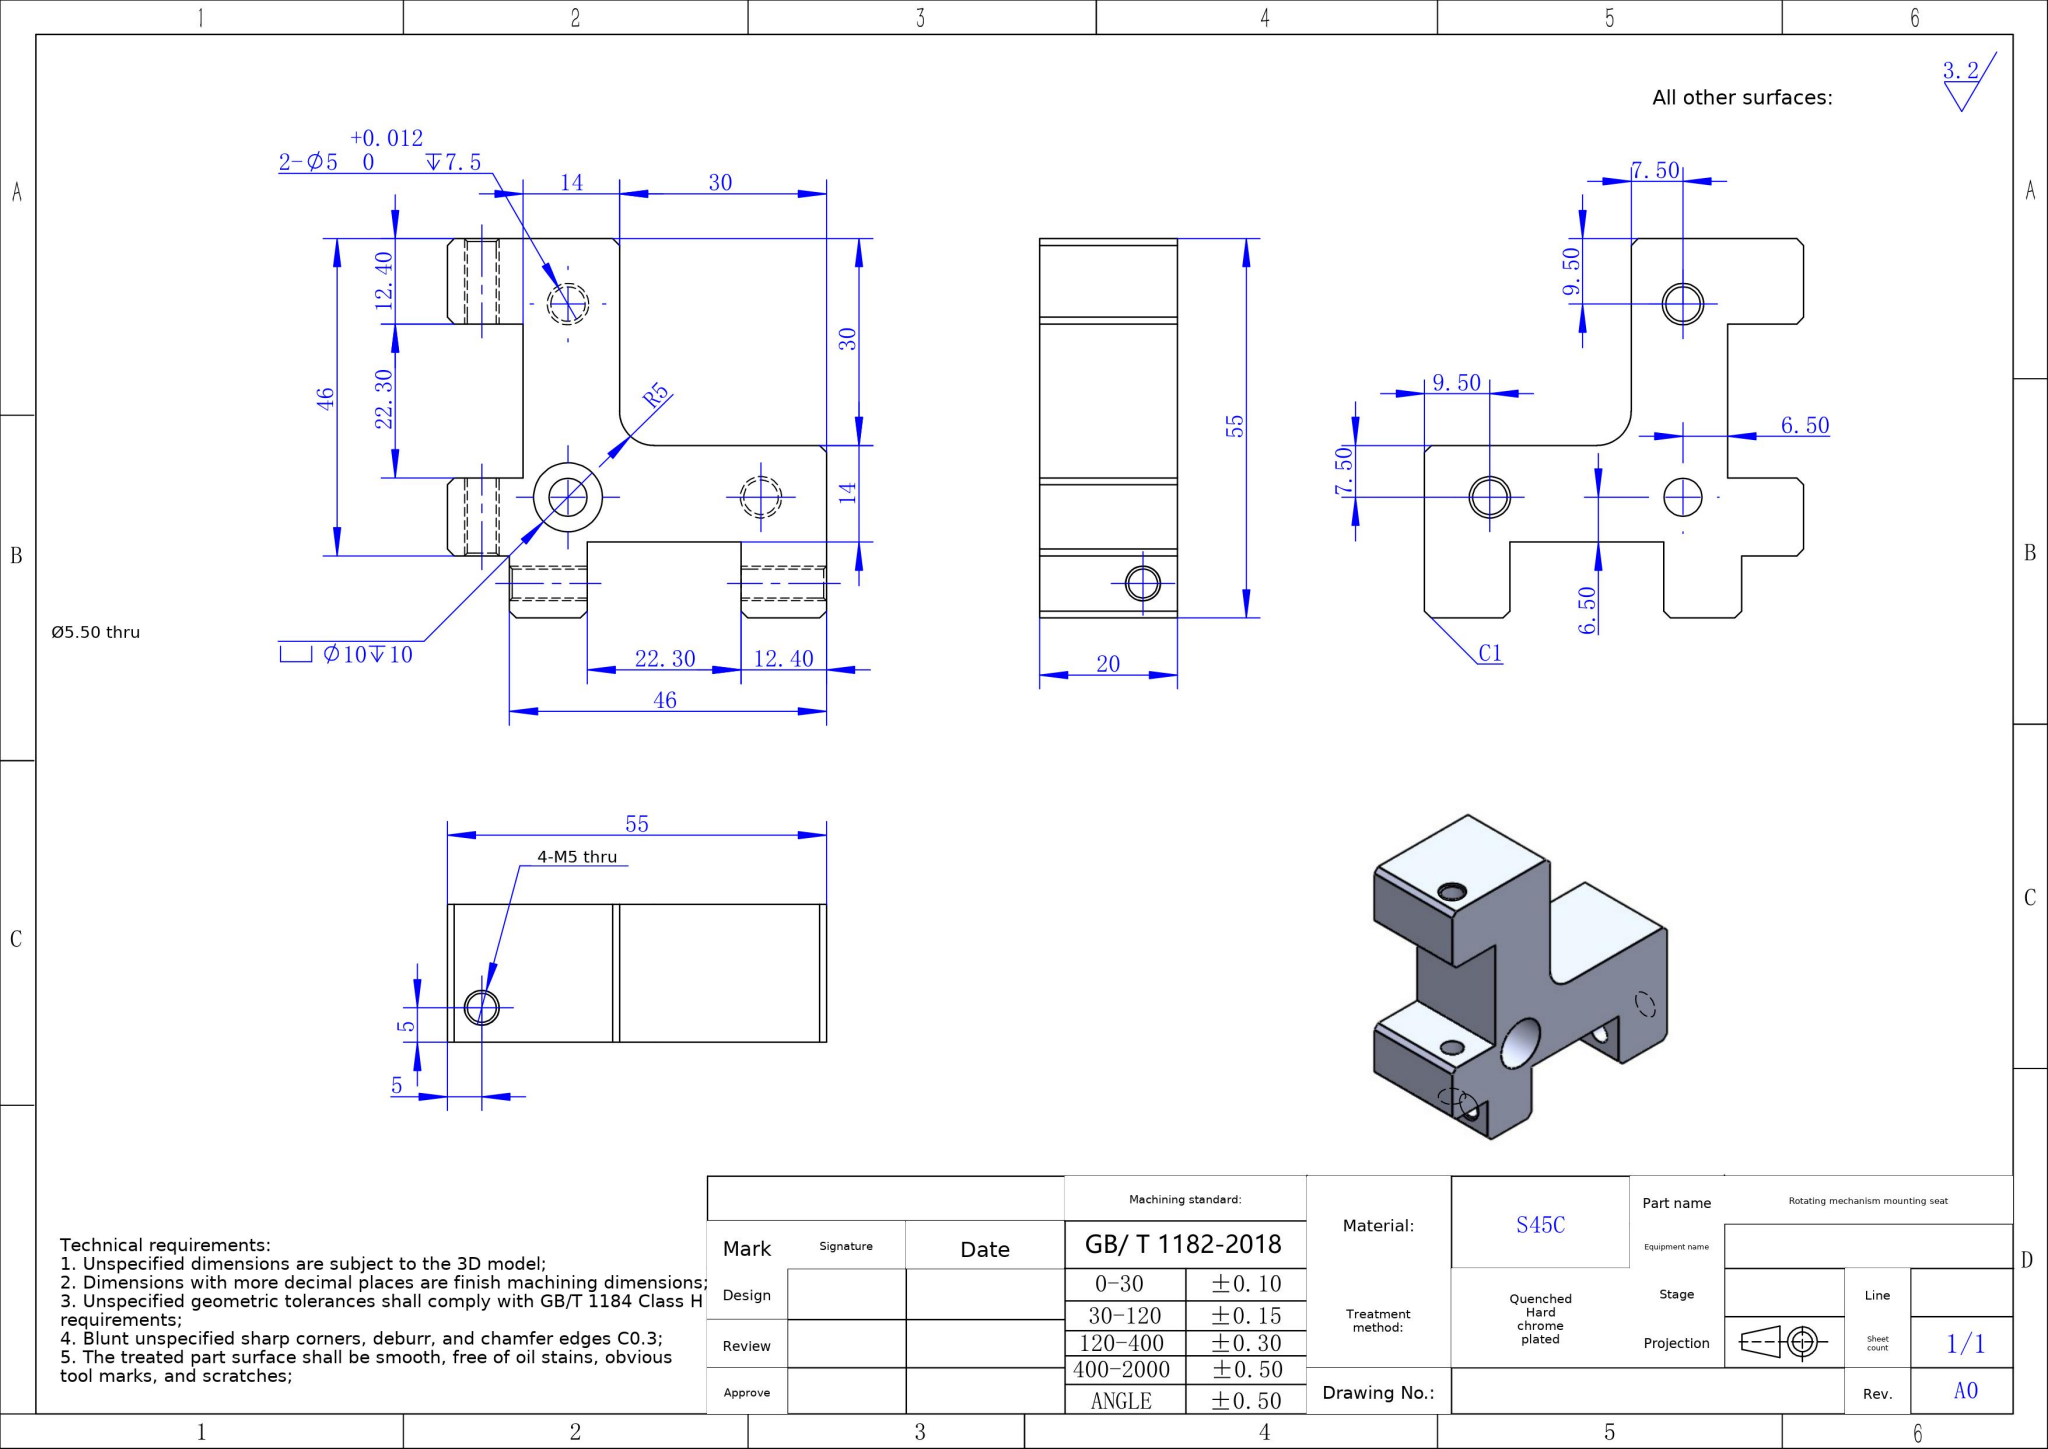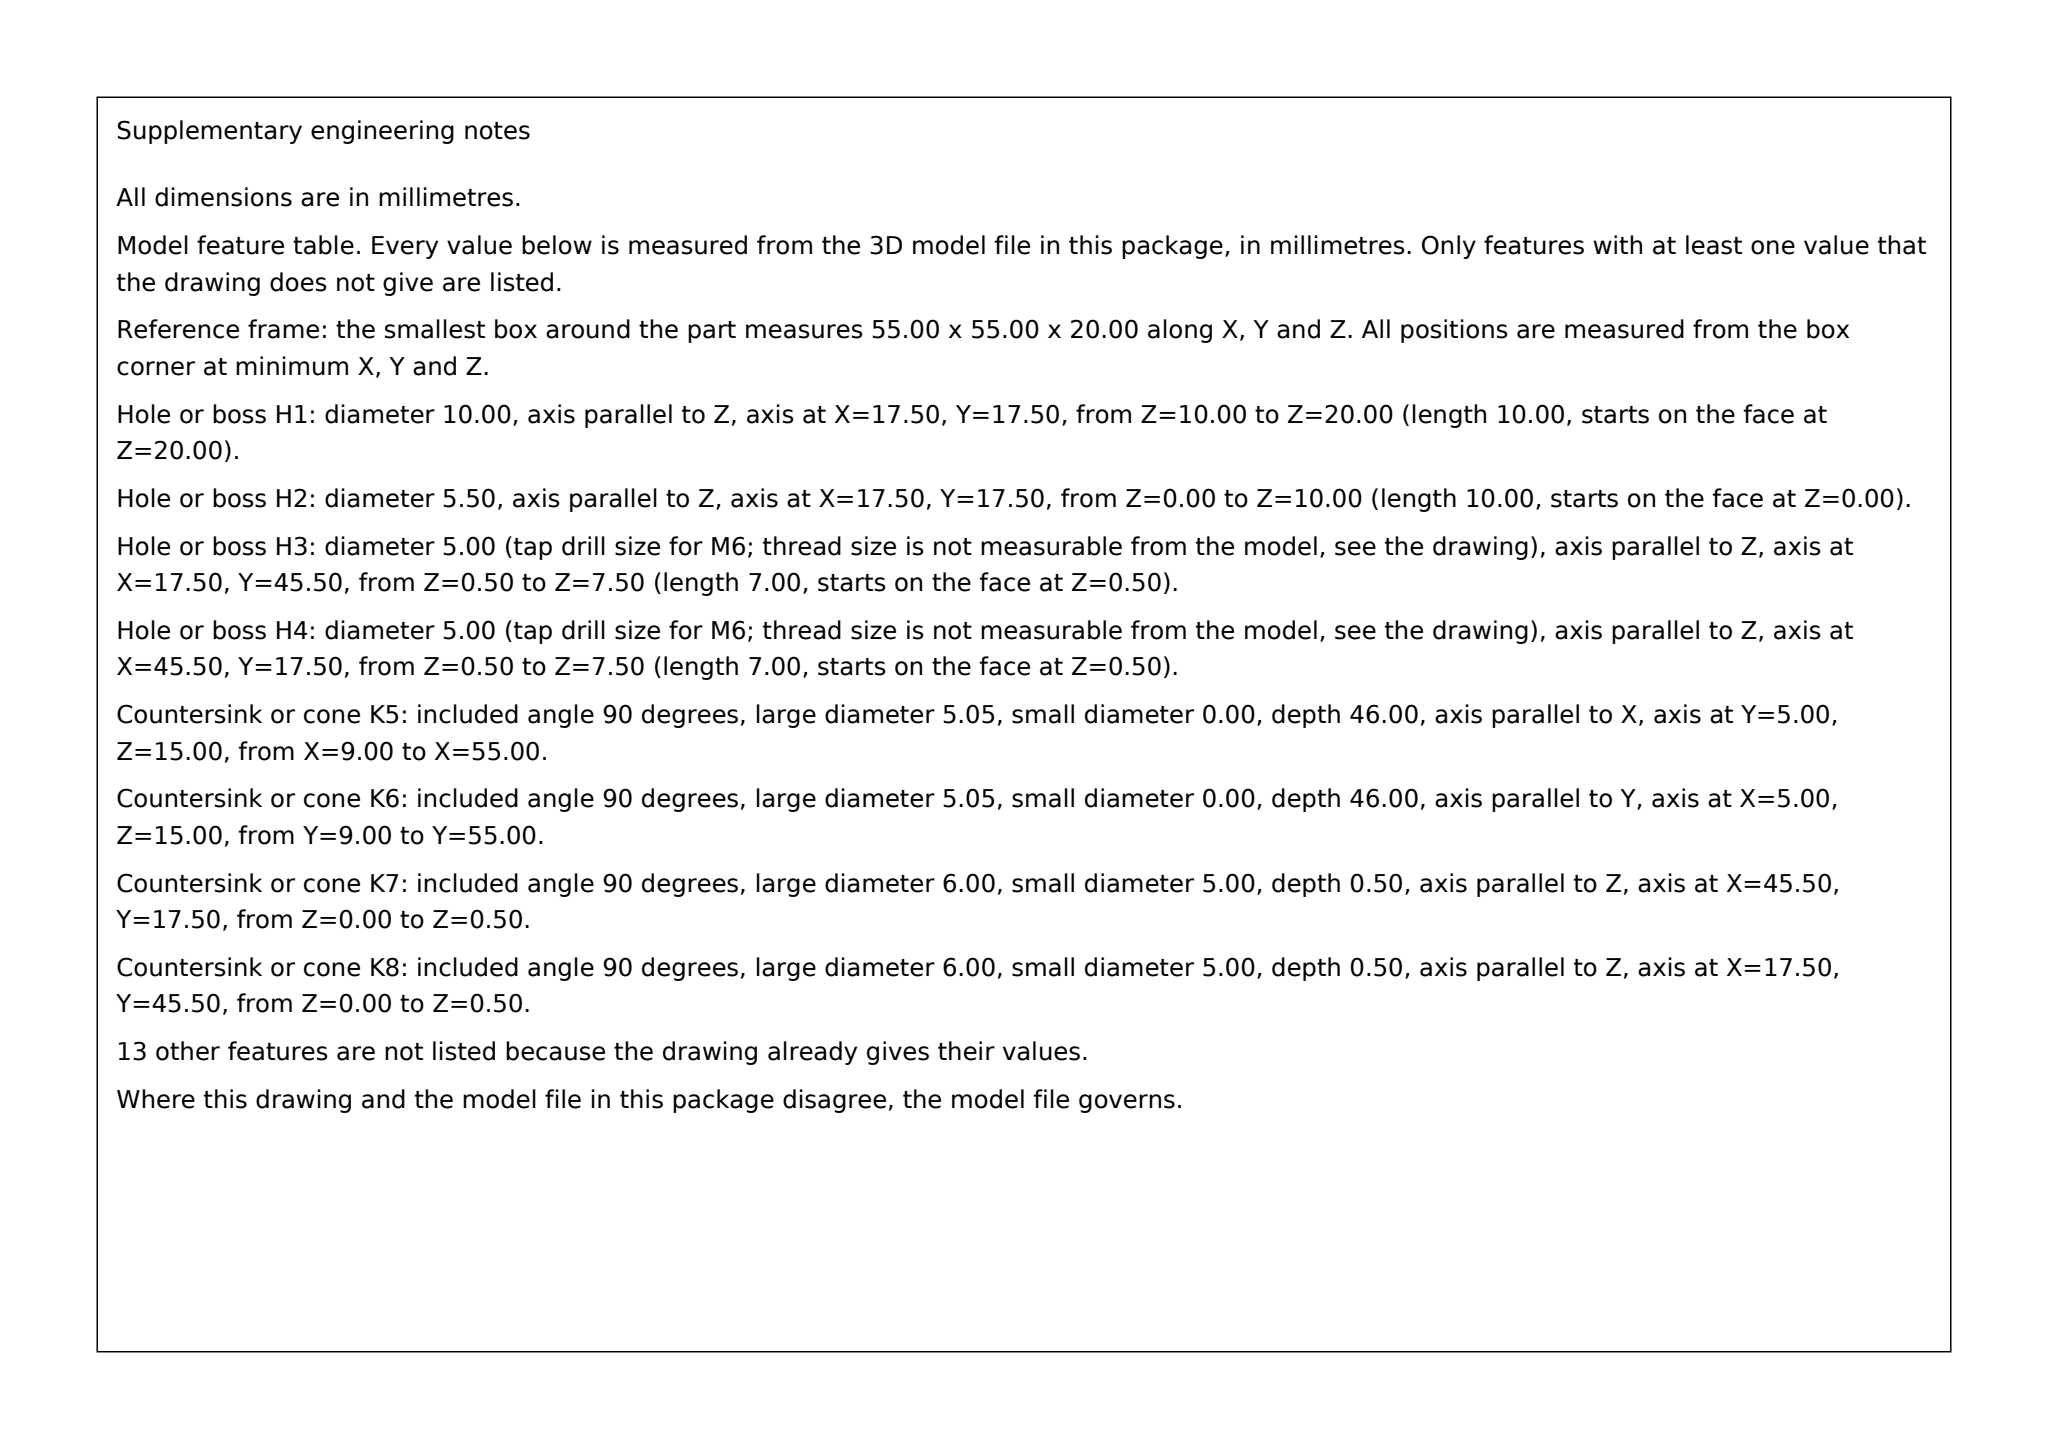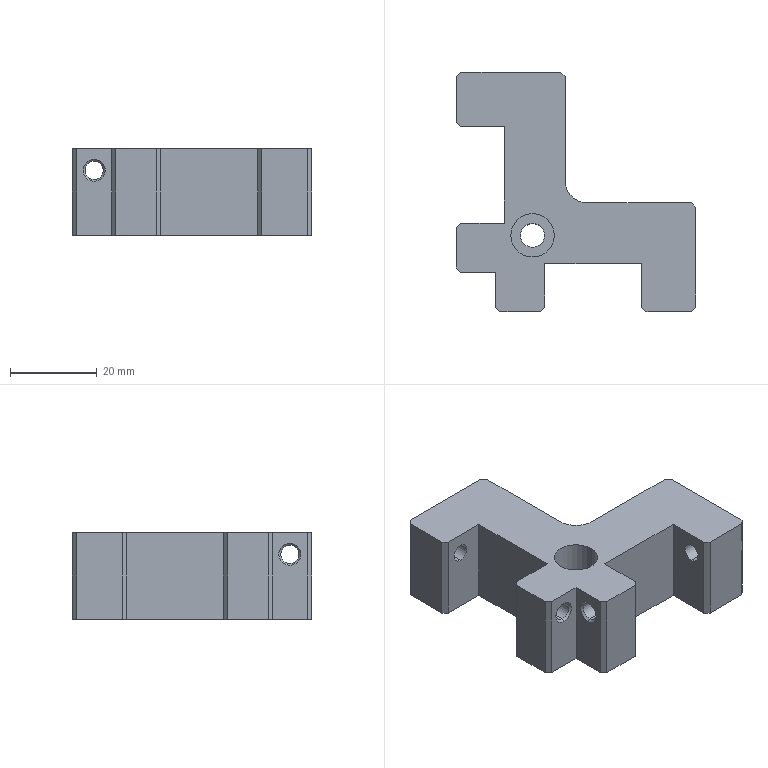Part | SolidWorks | mm | material S45C | 1 solid | 60 faces | box 55 x 55 x 20 mm | volume 29092 mm3 | plane 31 | cylinder 17 | cone 12 | commonest cylinder face diameters 4.2 x8 5 x4 10 x3 5.5 x2
build123d program:
from build123d import *

# Parameters (mm, degrees)
BOSS_EXTRUDE1_DEPTH         = 10
SKETCH2_R                   = 2.75
CUT_EXTRUDE1_DEPTH          = 20
SKETCH3_R                   = 5
CUT_EXTRUDE2_DEPTH          = 10
CHAMFER1_SIZE               = 1
M5_TAPPED_HOLE1_D           = 4.2
M5_TAPPED_HOLE1_DEPTH       = 17
M5_TAPPED_HOLE1_CSINK_D     = 5.05
M5_TAPPED_HOLE1_CSINK_ANGLE = 90
M5_TAPPED_HOLE1_TIP         = 1.262
M5_TAPPED_HOLE2_D           = 4.2
M5_TAPPED_HOLE2_DEPTH       = 17
M5_TAPPED_HOLE2_CSINK_D     = 5.05
M5_TAPPED_HOLE2_CSINK_ANGLE = 90
M5_TAPPED_HOLE2_TIP         = 1.262
M5_TAPPED_HOLE3_D           = 4.2
M5_TAPPED_HOLE3_DEPTH       = 17
M5_TAPPED_HOLE3_CSINK_D     = 5.05
M5_TAPPED_HOLE3_CSINK_ANGLE = 90
M5_TAPPED_HOLE3_TIP         = 1.262
M5_TAPPED_HOLE4_D           = 4.2
M5_TAPPED_HOLE4_DEPTH       = 17
M5_TAPPED_HOLE4_CSINK_D     = 5.05
M5_TAPPED_HOLE4_CSINK_ANGLE = 90
M5_TAPPED_HOLE4_TIP         = 1.262
SKETCH12_R                  = 2.5
CUT_EXTRUDE3_DEPTH          = 7.5
CHAMFER2_SIZE               = 0.5


with BuildPart() as part:
    # Sketch1 → Boss-Extrude1 (new, symmetric)
    with BuildSketch(Plane.XY):
        with BuildLine():
            Line((0, 0), (25, 0))
            Line((25, 0), (25, -25))
            ThreePointArc((25, -25), (26.464, -28.536), (30, -30))
            Line((30, -30), (55, -30))
            Line((55, -30), (55, -55))
            Line((55, -55), (42.6, -55))
            Line((42.6, -55), (42.6, -44))
            Line((42.6, -44), (20.3, -44))
            Line((20.3, -44), (20.3, -55))
            Line((20.3, -55), (9, -55))
            Line((9, -55), (9, -48.576))
            Line((9, -48.576), (9, -46))
            Line((9, -46), (0, -46))
            Line((0, -46), (0, -34.7))
            Line((0, -34.7), (11, -34.7))
            Line((11, -34.7), (11, -12.4))
            Line((11, -12.4), (0, -12.4))
            Line((0, -12.4), (0, 0))
        make_face()
    extrude(amount=BOSS_EXTRUDE1_DEPTH, both=True)

    # Sketch2 → Cut-Extrude1 (cut)
    with BuildSketch(Plane.XY.offset(10)):
        with Locations((17.5, -37.5)):
            Circle(SKETCH2_R)
    extrude(amount=-CUT_EXTRUDE1_DEPTH, mode=Mode.SUBTRACT)

    # Sketch3 → Cut-Extrude2 (cut)
    with BuildSketch(Plane.XY.offset(10)):
        with Locations((17.5, -37.5)):
            Circle(SKETCH3_R)
    extrude(amount=-CUT_EXTRUDE2_DEPTH, mode=Mode.SUBTRACT)

    # Chamfer1
    chamfer1_edges = [part.edges().sort_by_distance(p)[0] for p in [
        (0, 0, 0),
        (25, 0, 0),
        (55, -30, 0),
        (55, -55, 0),
        (42.6, -55, 0),
        (20.3, -55, 0),
        (9, -55, 0),
        (0, -46, 0),
        (0, -34.7, 0),
        (0, -12.4, 0),
    ]]
    chamfer(chamfer1_edges, length=CHAMFER1_SIZE)

    # M5 Tapped Hole1
    with Locations(Plane(origin=(0, 0, 0), x_dir=(1, 0, 0), z_dir=(0, 1, 0))):
        with Locations((5, -5)):
            CounterSinkHole(M5_TAPPED_HOLE1_D / 2, M5_TAPPED_HOLE1_CSINK_D / 2, depth=M5_TAPPED_HOLE1_DEPTH, counter_sink_angle=M5_TAPPED_HOLE1_CSINK_ANGLE)
            with Locations((0, 0, -(M5_TAPPED_HOLE1_DEPTH + M5_TAPPED_HOLE1_TIP / 2))):  # 118° drill point
                Cone(0, M5_TAPPED_HOLE1_D / 2, M5_TAPPED_HOLE1_TIP, mode=Mode.SUBTRACT)

    # M5 Tapped Hole2
    with Locations(Plane(origin=(0, -46, 0), x_dir=(-1, 0, 0), z_dir=(0, -1, 0))):
        with Locations((-5, -5)):
            CounterSinkHole(M5_TAPPED_HOLE2_D / 2, M5_TAPPED_HOLE2_CSINK_D / 2, depth=M5_TAPPED_HOLE2_DEPTH, counter_sink_angle=M5_TAPPED_HOLE2_CSINK_ANGLE)
            with Locations((0, 0, -(M5_TAPPED_HOLE2_DEPTH + M5_TAPPED_HOLE2_TIP / 2))):  # 118° drill point
                Cone(0, M5_TAPPED_HOLE2_D / 2, M5_TAPPED_HOLE2_TIP, mode=Mode.SUBTRACT)

    # M5 Tapped Hole3
    with Locations(Plane(origin=(55, 0, 0), x_dir=(0, 0, -1), z_dir=(1, 0, 0))):
        with Locations((-5, -50)):
            CounterSinkHole(M5_TAPPED_HOLE3_D / 2, M5_TAPPED_HOLE3_CSINK_D / 2, depth=M5_TAPPED_HOLE3_DEPTH, counter_sink_angle=M5_TAPPED_HOLE3_CSINK_ANGLE)
            with Locations((0, 0, -(M5_TAPPED_HOLE3_DEPTH + M5_TAPPED_HOLE3_TIP / 2))):  # 118° drill point
                Cone(0, M5_TAPPED_HOLE3_D / 2, M5_TAPPED_HOLE3_TIP, mode=Mode.SUBTRACT)

    # M5 Tapped Hole4
    with Locations(Plane.ZY.offset(-9)):
        with Locations((5, -50)):
            CounterSinkHole(M5_TAPPED_HOLE4_D / 2, M5_TAPPED_HOLE4_CSINK_D / 2, depth=M5_TAPPED_HOLE4_DEPTH, counter_sink_angle=M5_TAPPED_HOLE4_CSINK_ANGLE)
            with Locations((0, 0, -(M5_TAPPED_HOLE4_DEPTH + M5_TAPPED_HOLE4_TIP / 2))):  # 118° drill point
                Cone(0, M5_TAPPED_HOLE4_D / 2, M5_TAPPED_HOLE4_TIP, mode=Mode.SUBTRACT)

    # Sketch12 → Cut-Extrude3 (cut)
    with BuildSketch(Plane(origin=(0, 0, -10), x_dir=(-1, 0, 0), z_dir=(0, 0, -1))):
        with Locations((-45.5, -37.5)):
            Circle(SKETCH12_R)
        with Locations((-17.5, -9.5)):
            Circle(SKETCH12_R)
    extrude(amount=-CUT_EXTRUDE3_DEPTH, mode=Mode.SUBTRACT)

    # Chamfer2
    chamfer2_edges = [part.edges().sort_by_distance(p)[0] for p in [
        (48, -37.5, -10),
        (20, -9.5, -10),
    ]]
    chamfer(chamfer2_edges, length=CHAMFER2_SIZE)


solid = part.part